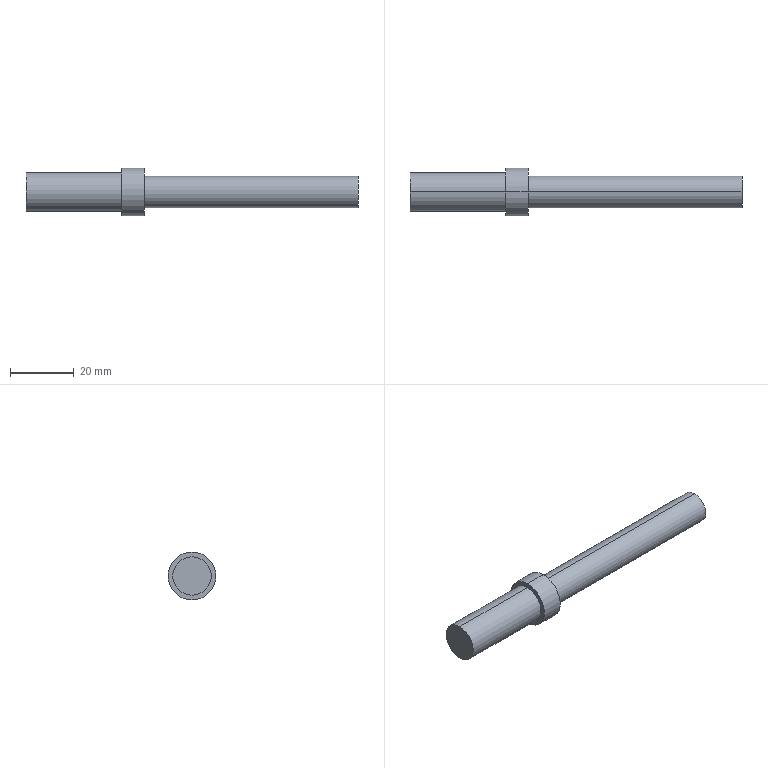Component | SolidWorks | -BeltTensionScrewRod-1 | 1 solid | 10 faces | box 104 x 15 x 15 mm | volume 9892 mm3 | cylinder 6 | plane 4 | commonest cylinder face diameters 12 x2 10 x2 15 x2
build123d program:
from build123d import *

# Parameters (mm, degrees)
SKETCH2_W           = 9.517
SKETCH2_H           = 20.387
CUT_EXTRUDE1_DEPTH  = 12
BOSS_EXTRUDE1_START = 22
SKETCH3_R           = 6
SKETCH3_R_2         = 5
BOSS_EXTRUDE1_DEPTH = 22
SKETCH4_R           = 7.5
BOSS_EXTRUDE2_DEPTH = 7
SKETCH5_R           = 9
SKETCH5_R_2         = 6
CUT_EXTRUDE2_DEPTH  = 90.906
SKETCH6_W           = 33.324
SKETCH6_H           = 24.059
CUT_EXTRUDE3_DEPTH  = 13.5


with BuildPart() as part:
    # Sketch1 → Revolve1 (revolve)
    with BuildSketch(Plane.XY, mode=Mode.PRIVATE) as revolve1_sk:
        Polygon((0, 0), (0, 5), (15, 5), (15, 6), (33, 6), (33, 9), (41, 9), (41, 5), (130, 5), (130, 0), align=None)
    revolve(revolve1_sk.sketch.rotate(Axis((-433.959, 0, 0), (1, 0, 0)), 90), axis=Axis((-433.959, 0, 0), (1, 0, 0)))

    # Sketch2 → Cut-Extrude1 (cut)
    with BuildSketch(Plane.ZY):
        with Locations((8.758, 1.458)):
            Rectangle(SKETCH2_W, SKETCH2_H)
    extrude(amount=-CUT_EXTRUDE1_DEPTH, mode=Mode.SUBTRACT)

    # Sketch3 → Boss-Extrude1 (add)
    with BuildSketch(Plane(origin=(41, 0, 0), x_dir=(0, 0, -1), z_dir=(1, 0, 0)).offset(BOSS_EXTRUDE1_START)):
        with Locations(Location((0, 0, 0), (0, 0, 180))):
            Circle(SKETCH3_R)
        with Locations(Location((0, 0, 0), (0, 0, 180))):
            Circle(SKETCH3_R_2, mode=Mode.SUBTRACT)
    extrude(amount=-BOSS_EXTRUDE1_DEPTH)

    # Sketch4 → Boss-Extrude2 (add)
    with BuildSketch(Plane(origin=(63, 0, 0), x_dir=(0, 0, -1), z_dir=(1, 0, 0))):
        Circle(SKETCH4_R)
    extrude(amount=-BOSS_EXTRUDE2_DEPTH)

    # Sketch5 → Cut-Extrude2 (cut, through all)
    with BuildSketch(Plane(origin=(41, 0, 0), x_dir=(0, 0, -1), z_dir=(1, 0, 0))):
        Circle(SKETCH5_R)
        with Locations(Location((0, 0, 0), (0, 0, 180))):
            Circle(SKETCH5_R_2, mode=Mode.SUBTRACT)
    extrude(amount=-CUT_EXTRUDE2_DEPTH, mode=Mode.SUBTRACT)

    # Sketch6 → Cut-Extrude3 (cut, symmetric)
    with BuildSketch(Plane.XY):
        with Locations((9.338, 0.5616)):
            Rectangle(SKETCH6_W, SKETCH6_H)
    extrude(amount=CUT_EXTRUDE3_DEPTH, both=True, mode=Mode.SUBTRACT)


solid = part.part

# Placed as in the assembly
solid = solid.moved(Location((-316, 1094.5, -20), (0, 0, 0)))
STEP:
#1=COLOUR_RGB('',0.7922,0.8196,0.9333);
#2=FILL_AREA_STYLE_COLOUR('',#1);
#3=FILL_AREA_STYLE('',(#2));
#4=SURFACE_STYLE_FILL_AREA(#3);
#5=SURFACE_SIDE_STYLE('',(#4));
#6=SURFACE_STYLE_USAGE(.BOTH.,#5);
#7=PRESENTATION_STYLE_ASSIGNMENT((#6));
#8=CARTESIAN_POINT('',(-10.236,43.091,-1.024));
#9=VERTEX_POINT('',#8);
#10=CARTESIAN_POINT('',(-10.236,43.091,-0.5512));
#11=VERTEX_POINT('',#10);
#12=CARTESIAN_POINT('',(-10.236,43.091,-0.7874));
#13=DIRECTION('',(1.,0.,0.));
#14=DIRECTION('',(0.,0.,-1.));
#15=AXIS2_PLACEMENT_3D('',#12,#13,#14);
#16=CIRCLE('',#15,0.2362);
#17=EDGE_CURVE('',#9,#11,#16,.T.);
#18=ORIENTED_EDGE('',*,*,#17,.F.);
#19=CARTESIAN_POINT('',(-11.417,43.091,-1.024));
#20=VERTEX_POINT('',#19);
#21=CARTESIAN_POINT('',(-29.526,43.091,-1.024));
#22=DIRECTION('',(-1.,0.,0.));
#23=VECTOR('',#22,39.37);
#24=LINE('',#21,#23);
#25=EDGE_CURVE('',#9,#20,#24,.T.);
#26=ORIENTED_EDGE('',*,*,#25,.T.);
#27=CARTESIAN_POINT('',(-11.417,43.091,-0.5512));
#28=VERTEX_POINT('',#27);
#29=CARTESIAN_POINT('',(-11.417,43.091,-0.7874));
#30=DIRECTION('',(1.,0.,0.));
#31=DIRECTION('',(0.,1.,0.));
#32=AXIS2_PLACEMENT_3D('',#29,#30,#31);
#33=CIRCLE('',#32,0.2362);
#34=EDGE_CURVE('',#20,#28,#33,.T.);
#35=ORIENTED_EDGE('',*,*,#34,.T.);
#36=CARTESIAN_POINT('',(-29.526,43.091,-0.5512));
#37=DIRECTION('',(-1.,0.,0.));
#38=VECTOR('',#37,39.37);
#39=LINE('',#36,#38);
#40=EDGE_CURVE('',#11,#28,#39,.T.);
#41=ORIENTED_EDGE('',*,*,#40,.F.);
#42=EDGE_LOOP('',(#18,#26,#35,#41));
#43=FACE_OUTER_BOUND('',#42,.T.);
#44=CARTESIAN_POINT('',(-29.526,43.091,-0.7874));
#45=DIRECTION('',(-1.,0.,0.));
#46=DIRECTION('',(0.,0.,1.));
#47=AXIS2_PLACEMENT_3D('',#44,#45,#46);
#48=CYLINDRICAL_SURFACE('',#47,0.2362);
#49=ADVANCED_FACE('',(#43),#48,.T.);
#50=CARTESIAN_POINT('',(-7.323,43.091,-0.5906));
#51=VERTEX_POINT('',#50);
#52=CARTESIAN_POINT('',(-7.323,43.091,-0.9843));
#53=VERTEX_POINT('',#52);
#54=CARTESIAN_POINT('',(-7.323,43.091,-0.7874));
#55=DIRECTION('',(-1.,0.,0.));
#56=DIRECTION('',(0.,0.,1.));
#57=AXIS2_PLACEMENT_3D('',#54,#55,#56);
#58=CIRCLE('',#57,0.1969);
#59=EDGE_CURVE('',#51,#53,#58,.T.);
#60=ORIENTED_EDGE('',*,*,#59,.T.);
#61=CARTESIAN_POINT('',(-9.961,43.091,-0.9843));
#62=VERTEX_POINT('',#61);
#63=CARTESIAN_POINT('',(-29.526,43.091,-0.9843));
#64=DIRECTION('',(-1.,0.,0.));
#65=VECTOR('',#64,39.37);
#66=LINE('',#63,#65);
#67=EDGE_CURVE('',#53,#62,#66,.T.);
#68=ORIENTED_EDGE('',*,*,#67,.T.);
#69=CARTESIAN_POINT('',(-9.961,43.091,-0.5906));
#70=VERTEX_POINT('',#69);
#71=CARTESIAN_POINT('',(-9.961,43.091,-0.7874));
#72=DIRECTION('',(1.,0.,0.));
#73=DIRECTION('',(0.,0.,-1.));
#74=AXIS2_PLACEMENT_3D('',#71,#72,#73);
#75=CIRCLE('',#74,0.1969);
#76=EDGE_CURVE('',#62,#70,#75,.T.);
#77=ORIENTED_EDGE('',*,*,#76,.T.);
#78=CARTESIAN_POINT('',(-29.526,43.091,-0.5906));
#79=DIRECTION('',(-1.,0.,0.));
#80=VECTOR('',#79,39.37);
#81=LINE('',#78,#80);
#82=EDGE_CURVE('',#51,#70,#81,.T.);
#83=ORIENTED_EDGE('',*,*,#82,.F.);
#84=EDGE_LOOP('',(#60,#68,#77,#83));
#85=FACE_OUTER_BOUND('',#84,.T.);
#86=CARTESIAN_POINT('',(-29.526,43.091,-0.7874));
#87=DIRECTION('',(-1.,0.,0.));
#88=DIRECTION('',(0.,0.,1.));
#89=AXIS2_PLACEMENT_3D('',#86,#87,#88);
#90=CYLINDRICAL_SURFACE('',#89,0.1969);
#91=ADVANCED_FACE('',(#85),#90,.T.);
#92=CARTESIAN_POINT('',(-10.236,43.091,-1.083));
#93=VERTEX_POINT('',#92);
#94=CARTESIAN_POINT('',(-10.236,43.091,-0.4921));
#95=VERTEX_POINT('',#94);
#96=CARTESIAN_POINT('',(-10.236,43.091,-0.7874));
#97=DIRECTION('',(1.,0.,0.));
#98=DIRECTION('',(0.,0.,-1.));
#99=AXIS2_PLACEMENT_3D('',#96,#97,#98);
#100=CIRCLE('',#99,0.2953);
#101=EDGE_CURVE('',#93,#95,#100,.T.);
#102=ORIENTED_EDGE('',*,*,#101,.T.);
#103=CARTESIAN_POINT('',(-9.961,43.091,-0.4921));
#104=VERTEX_POINT('',#103);
#105=CARTESIAN_POINT('',(-10.236,43.091,-0.4921));
#106=DIRECTION('',(1.,0.,0.));
#107=VECTOR('',#106,39.37);
#108=LINE('',#105,#107);
#109=EDGE_CURVE('',#95,#104,#108,.T.);
#110=ORIENTED_EDGE('',*,*,#109,.T.);
#111=CARTESIAN_POINT('',(-9.961,43.091,-1.083));
#112=VERTEX_POINT('',#111);
#113=CARTESIAN_POINT('',(-9.961,43.091,-0.7874));
#114=DIRECTION('',(1.,0.,0.));
#115=DIRECTION('',(0.,0.,-1.));
#116=AXIS2_PLACEMENT_3D('',#113,#114,#115);
#117=CIRCLE('',#116,0.2953);
#118=EDGE_CURVE('',#112,#104,#117,.T.);
#119=ORIENTED_EDGE('',*,*,#118,.F.);
#120=CARTESIAN_POINT('',(-10.236,43.091,-1.083));
#121=DIRECTION('',(1.,0.,0.));
#122=VECTOR('',#121,39.37);
#123=LINE('',#120,#122);
#124=EDGE_CURVE('',#93,#112,#123,.T.);
#125=ORIENTED_EDGE('',*,*,#124,.F.);
#126=EDGE_LOOP('',(#102,#110,#119,#125));
#127=FACE_OUTER_BOUND('',#126,.T.);
#128=CARTESIAN_POINT('',(-10.236,43.091,-0.7874));
#129=DIRECTION('',(1.,0.,0.));
#130=DIRECTION('',(0.,0.,-1.));
#131=AXIS2_PLACEMENT_3D('',#128,#129,#130);
#132=CYLINDRICAL_SURFACE('',#131,0.2953);
#133=ADVANCED_FACE('',(#127),#132,.T.);
#134=ORIENTED_EDGE('',*,*,#101,.F.);
#135=CARTESIAN_POINT('',(-10.236,43.091,-0.7874));
#136=DIRECTION('',(1.,0.,0.));
#137=DIRECTION('',(0.,0.,-1.));
#138=AXIS2_PLACEMENT_3D('',#135,#136,#137);
#139=CIRCLE('',#138,0.2953);
#140=EDGE_CURVE('',#95,#93,#139,.T.);
#141=ORIENTED_EDGE('',*,*,#140,.F.);
#142=EDGE_LOOP('',(#134,#141));
#143=FACE_OUTER_BOUND('',#142,.T.);
#144=CARTESIAN_POINT('',(-10.236,43.091,-0.7874));
#145=DIRECTION('',(1.,0.,0.));
#146=DIRECTION('',(0.,0.,-1.));
#147=AXIS2_PLACEMENT_3D('',#144,#145,#146);
#148=CIRCLE('',#147,0.2362);
#149=EDGE_CURVE('',#11,#9,#148,.T.);
#150=ORIENTED_EDGE('',*,*,#149,.T.);
#151=ORIENTED_EDGE('',*,*,#17,.T.);
#152=EDGE_LOOP('',(#150,#151));
#153=FACE_BOUND('',#152,.T.);
#154=CARTESIAN_POINT('',(-10.236,43.091,-0.7874));
#155=DIRECTION('',(1.,0.,0.));
#156=DIRECTION('',(0.,0.,-1.));
#157=AXIS2_PLACEMENT_3D('',#154,#155,#156);
#158=PLANE('',#157);
#159=ADVANCED_FACE('',(#143,#153),#158,.F.);
#160=ORIENTED_EDGE('',*,*,#109,.F.);
#161=ORIENTED_EDGE('',*,*,#140,.T.);
#162=ORIENTED_EDGE('',*,*,#124,.T.);
#163=CARTESIAN_POINT('',(-9.961,43.091,-0.7874));
#164=DIRECTION('',(1.,0.,0.));
#165=DIRECTION('',(0.,0.,-1.));
#166=AXIS2_PLACEMENT_3D('',#163,#164,#165);
#167=CIRCLE('',#166,0.2953);
#168=EDGE_CURVE('',#104,#112,#167,.T.);
#169=ORIENTED_EDGE('',*,*,#168,.F.);
#170=EDGE_LOOP('',(#160,#161,#162,#169));
#171=FACE_OUTER_BOUND('',#170,.T.);
#172=CARTESIAN_POINT('',(-10.236,43.091,-0.7874));
#173=DIRECTION('',(1.,0.,0.));
#174=DIRECTION('',(0.,0.,-1.));
#175=AXIS2_PLACEMENT_3D('',#172,#173,#174);
#176=CYLINDRICAL_SURFACE('',#175,0.2953);
#177=ADVANCED_FACE('',(#171),#176,.T.);
#178=ORIENTED_EDGE('',*,*,#59,.F.);
#179=CARTESIAN_POINT('',(-7.323,43.091,-0.7874));
#180=DIRECTION('',(-1.,0.,0.));
#181=DIRECTION('',(0.,0.,1.));
#182=AXIS2_PLACEMENT_3D('',#179,#180,#181);
#183=CIRCLE('',#182,0.1969);
#184=EDGE_CURVE('',#53,#51,#183,.T.);
#185=ORIENTED_EDGE('',*,*,#184,.F.);
#186=EDGE_LOOP('',(#178,#185));
#187=FACE_OUTER_BOUND('',#186,.T.);
#188=CARTESIAN_POINT('',(-7.323,43.287,-0.7874));
#189=DIRECTION('',(-1.,0.,0.));
#190=DIRECTION('',(0.,0.,1.));
#191=AXIS2_PLACEMENT_3D('',#188,#189,#190);
#192=PLANE('',#191);
#193=ADVANCED_FACE('',(#187),#192,.F.);
#194=ORIENTED_EDGE('',*,*,#67,.F.);
#195=ORIENTED_EDGE('',*,*,#184,.T.);
#196=ORIENTED_EDGE('',*,*,#82,.T.);
#197=CARTESIAN_POINT('',(-9.961,43.091,-0.7874));
#198=DIRECTION('',(1.,0.,0.));
#199=DIRECTION('',(0.,0.,-1.));
#200=AXIS2_PLACEMENT_3D('',#197,#198,#199);
#201=CIRCLE('',#200,0.1969);
#202=EDGE_CURVE('',#70,#62,#201,.T.);
#203=ORIENTED_EDGE('',*,*,#202,.T.);
#204=EDGE_LOOP('',(#194,#195,#196,#203));
#205=FACE_OUTER_BOUND('',#204,.T.);
#206=CARTESIAN_POINT('',(-29.526,43.091,-0.7874));
#207=DIRECTION('',(-1.,0.,0.));
#208=DIRECTION('',(0.,0.,1.));
#209=AXIS2_PLACEMENT_3D('',#206,#207,#208);
#210=CYLINDRICAL_SURFACE('',#209,0.1969);
#211=ADVANCED_FACE('',(#205),#210,.T.);
#212=ORIENTED_EDGE('',*,*,#202,.F.);
#213=ORIENTED_EDGE('',*,*,#76,.F.);
#214=EDGE_LOOP('',(#212,#213));
#215=FACE_BOUND('',#214,.T.);
#216=ORIENTED_EDGE('',*,*,#118,.T.);
#217=ORIENTED_EDGE('',*,*,#168,.T.);
#218=EDGE_LOOP('',(#216,#217));
#219=FACE_OUTER_BOUND('',#218,.T.);
#220=CARTESIAN_POINT('',(-9.961,43.091,-0.7874));
#221=DIRECTION('',(1.,0.,0.));
#222=DIRECTION('',(0.,0.,-1.));
#223=AXIS2_PLACEMENT_3D('',#220,#221,#222);
#224=PLANE('',#223);
#225=ADVANCED_FACE('',(#215,#219),#224,.T.);
#226=ORIENTED_EDGE('',*,*,#25,.F.);
#227=ORIENTED_EDGE('',*,*,#149,.F.);
#228=ORIENTED_EDGE('',*,*,#40,.T.);
#229=CARTESIAN_POINT('',(-11.417,43.091,-0.7874));
#230=DIRECTION('',(1.,0.,0.));
#231=DIRECTION('',(0.,1.,0.));
#232=AXIS2_PLACEMENT_3D('',#229,#230,#231);
#233=CIRCLE('',#232,0.2362);
#234=EDGE_CURVE('',#28,#20,#233,.T.);
#235=ORIENTED_EDGE('',*,*,#234,.T.);
#236=EDGE_LOOP('',(#226,#227,#228,#235));
#237=FACE_OUTER_BOUND('',#236,.T.);
#238=CARTESIAN_POINT('',(-29.526,43.091,-0.7874));
#239=DIRECTION('',(-1.,0.,0.));
#240=DIRECTION('',(0.,0.,1.));
#241=AXIS2_PLACEMENT_3D('',#238,#239,#240);
#242=CYLINDRICAL_SURFACE('',#241,0.2362);
#243=ADVANCED_FACE('',(#237),#242,.T.);
#244=ORIENTED_EDGE('',*,*,#234,.F.);
#245=ORIENTED_EDGE('',*,*,#34,.F.);
#246=EDGE_LOOP('',(#244,#245));
#247=FACE_OUTER_BOUND('',#246,.T.);
#248=CARTESIAN_POINT('',(-11.417,43.586,-1.319));
#249=DIRECTION('',(1.,0.,0.));
#250=DIRECTION('',(-0.,1.,0.));
#251=AXIS2_PLACEMENT_3D('',#248,#249,#250);
#252=PLANE('',#251);
#253=ADVANCED_FACE('',(#247),#252,.F.);
#254=CLOSED_SHELL('',(#49,#91,#133,#159,#177,#193,#211,#225,#243,#253));
#255=MANIFOLD_SOLID_BREP('',#254);
#256=STYLED_ITEM('',(#7),#255);
#257=PRESENTATION_LAYER_ASSIGNMENT('','',(#256));
#258=(LENGTH_UNIT()NAMED_UNIT(*)SI_UNIT($,.METRE.));
#259=LENGTH_MEASURE_WITH_UNIT(LENGTH_MEASURE(0.0254),#258);
#260=DIMENSIONAL_EXPONENTS(1.,0.,0.,0.,0.,0.,0.);
#261=(CONVERSION_BASED_UNIT('',#259)LENGTH_UNIT()NAMED_UNIT(#260));
#262=UNCERTAINTY_MEASURE_WITH_UNIT(LENGTH_MEASURE(0.00001),#261,'','');
#263=(NAMED_UNIT(*)PLANE_ANGLE_UNIT()SI_UNIT($,.RADIAN.));
#264=(NAMED_UNIT(*)SI_UNIT($,.STERADIAN.)SOLID_ANGLE_UNIT());
#265=(GEOMETRIC_REPRESENTATION_CONTEXT(3)GLOBAL_UNCERTAINTY_ASSIGNED_CONTEXT((#262))GLOBAL_UNIT_ASSIGNED_CONTEXT((#261,#263,#264))REPRESENTATION_CONTEXT('',''));
#266=MECHANICAL_DESIGN_GEOMETRIC_PRESENTATION_REPRESENTATION('',(#256),#265);
#267=CARTESIAN_POINT('',(0.,0.,0.));
#268=DIRECTION('',(0.,0.,1.));
#269=DIRECTION('',(1.,0.,0.));
#270=AXIS2_PLACEMENT_3D('',#267,#268,#269);
#271=(LENGTH_UNIT()NAMED_UNIT(*)SI_UNIT($,.METRE.));
#272=LENGTH_MEASURE_WITH_UNIT(LENGTH_MEASURE(0.0254),#271);
#273=DIMENSIONAL_EXPONENTS(1.,0.,0.,0.,0.,0.,0.);
#274=(CONVERSION_BASED_UNIT('',#272)LENGTH_UNIT()NAMED_UNIT(#273));
#275=UNCERTAINTY_MEASURE_WITH_UNIT(LENGTH_MEASURE(0.00001),#274,'','');
#276=(NAMED_UNIT(*)PLANE_ANGLE_UNIT()SI_UNIT($,.RADIAN.));
#277=(NAMED_UNIT(*)SI_UNIT($,.STERADIAN.)SOLID_ANGLE_UNIT());
#278=(GEOMETRIC_REPRESENTATION_CONTEXT(3)GLOBAL_UNCERTAINTY_ASSIGNED_CONTEXT((#275))GLOBAL_UNIT_ASSIGNED_CONTEXT((#274,#276,#277))REPRESENTATION_CONTEXT('',''));
#279=ADVANCED_BREP_SHAPE_REPRESENTATION('',(#255,#270),#278);